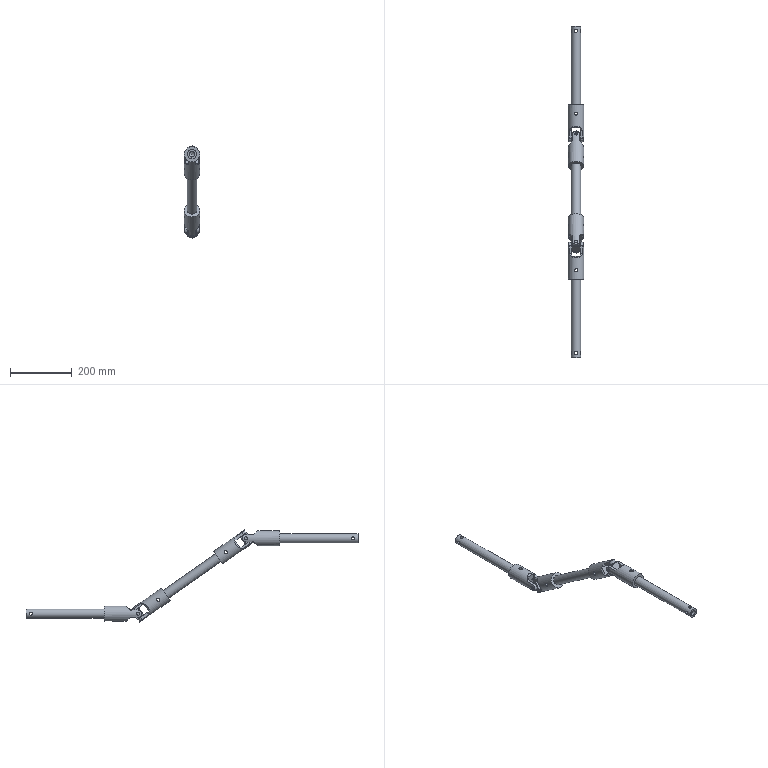Assembly | NX | mm | 9 component files | 9 solids | 140 faces | box 50 x 1074.96 x 297.92 mm | volume 936973 mm3 | cylinder 70 | plane 66 | cone 4 | commonest cylinder face diameters 10 x40 22 x8 11 x8 30 x7 50 x4 18 x3
Bill of materials:
unnamed part 1 | 2 |  | Block shaped like a cube or rectangular prism, with cylindrical pins sticking out along two perpendicular axes. One pair of pins comes out of opposite faces on one axis. A second pair comes out of the other two opposite faces on a perpendicular axis. Overall it forms a cross-shaped block with pins.
unnamed part 2 | 4 |  | Cylindrical body with a fork (clevis-like) at one end. Two flat, parallel tangs with rounded ends stick out from the body, with an open slot between them. Each tang has a transverse hole near its end, and the holes line up. The cylinder narrows to the tangs through angled transitions. The slot ends inside the body with a curved bottom. One radial through-hole crosses the cylindrical body nearer the other end, which looks closed and flat.
unnamed part 3 | 3 |  | Long, straight, thin-walled round tube with a concentric through-bore. Each end has transverse cross-holes through the wall. They appear to run in two perpendicular directions at each end.
Mates:
1. fix | universal_joint_connector_model1 4 component
2. touch align | connecting_rod_model1 3 face | universal_joint_connector_model1 4 face
3. touch align | universal_joint_center_block_model1 2 face | universal_joint_connector_model1 4 face
4. center | universal_joint_center_block_model1 2 face | universal_joint_center_block_model1 2 face | universal_joint_connector_model1 4 face | universal_joint_connector_model1 4 face
5. touch align | universal_joint_connector_model1 3 face | universal_joint_center_block_model1 2 face
6. center | universal_joint_connector_model1 3 face | universal_joint_connector_model1 3 face | universal_joint_center_block_model1 2 face | universal_joint_center_block_model1 2 face
7. touch align | connecting_rod_model1 2 face | universal_joint_connector_model1 3 face
8. touch align | connecting_rod_model1 2 face | universal_joint_connector_model1 3 face
9. parallel | universal_joint_connector_model1 3 face | universal_joint_center_block_model1 2 face
10. touch align | universal_joint_center_block_model1 1 face | universal_joint_connector_model1 2 face
11. center | universal_joint_center_block_model1 1 face | universal_joint_center_block_model1 1 face | universal_joint_connector_model1 2 face | universal_joint_connector_model1 2 face
12. touch align | universal_joint_connector_model1 2 face | connecting_rod_model1 2 face
13. touch align | universal_joint_connector_model1 2 face | connecting_rod_model1 2 face
14. parallel | universal_joint_center_block_model1 1 face | universal_joint_connector_model1 2 face
15. touch align | universal_joint_connector_model1 1 face | universal_joint_center_block_model1 1 face
16. center | universal_joint_connector_model1 1 face | universal_joint_connector_model1 1 face | universal_joint_center_block_model1 1 face | universal_joint_center_block_model1 1 face
17. touch align | connecting_rod_model1 1 face | universal_joint_connector_model1 1 face
18. touch align | connecting_rod_model1 1 face | universal_joint_connector_model1 1 face
19. parallel | connecting_rod_model1 3 face | connecting_rod_model1 1 face